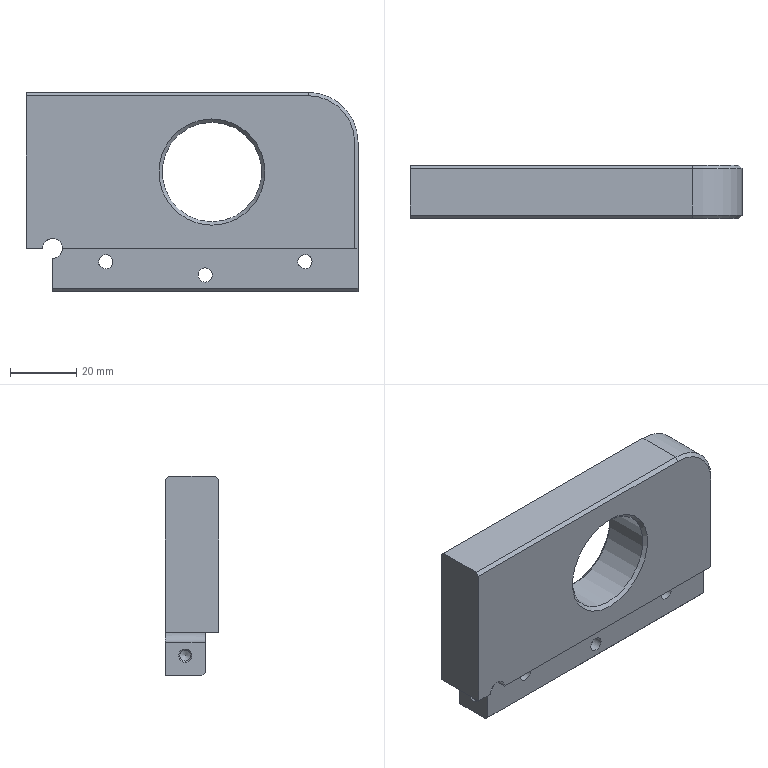Component | NX | RIGHT_PLATE | 1 solid | 43 faces | volume 75259 mm3 | plane 18 | cylinder 13 | cone 12 | commonest cylinder face diameters 3.3 x4 4.3 x3 7.5 x3 30 x2 6 x1